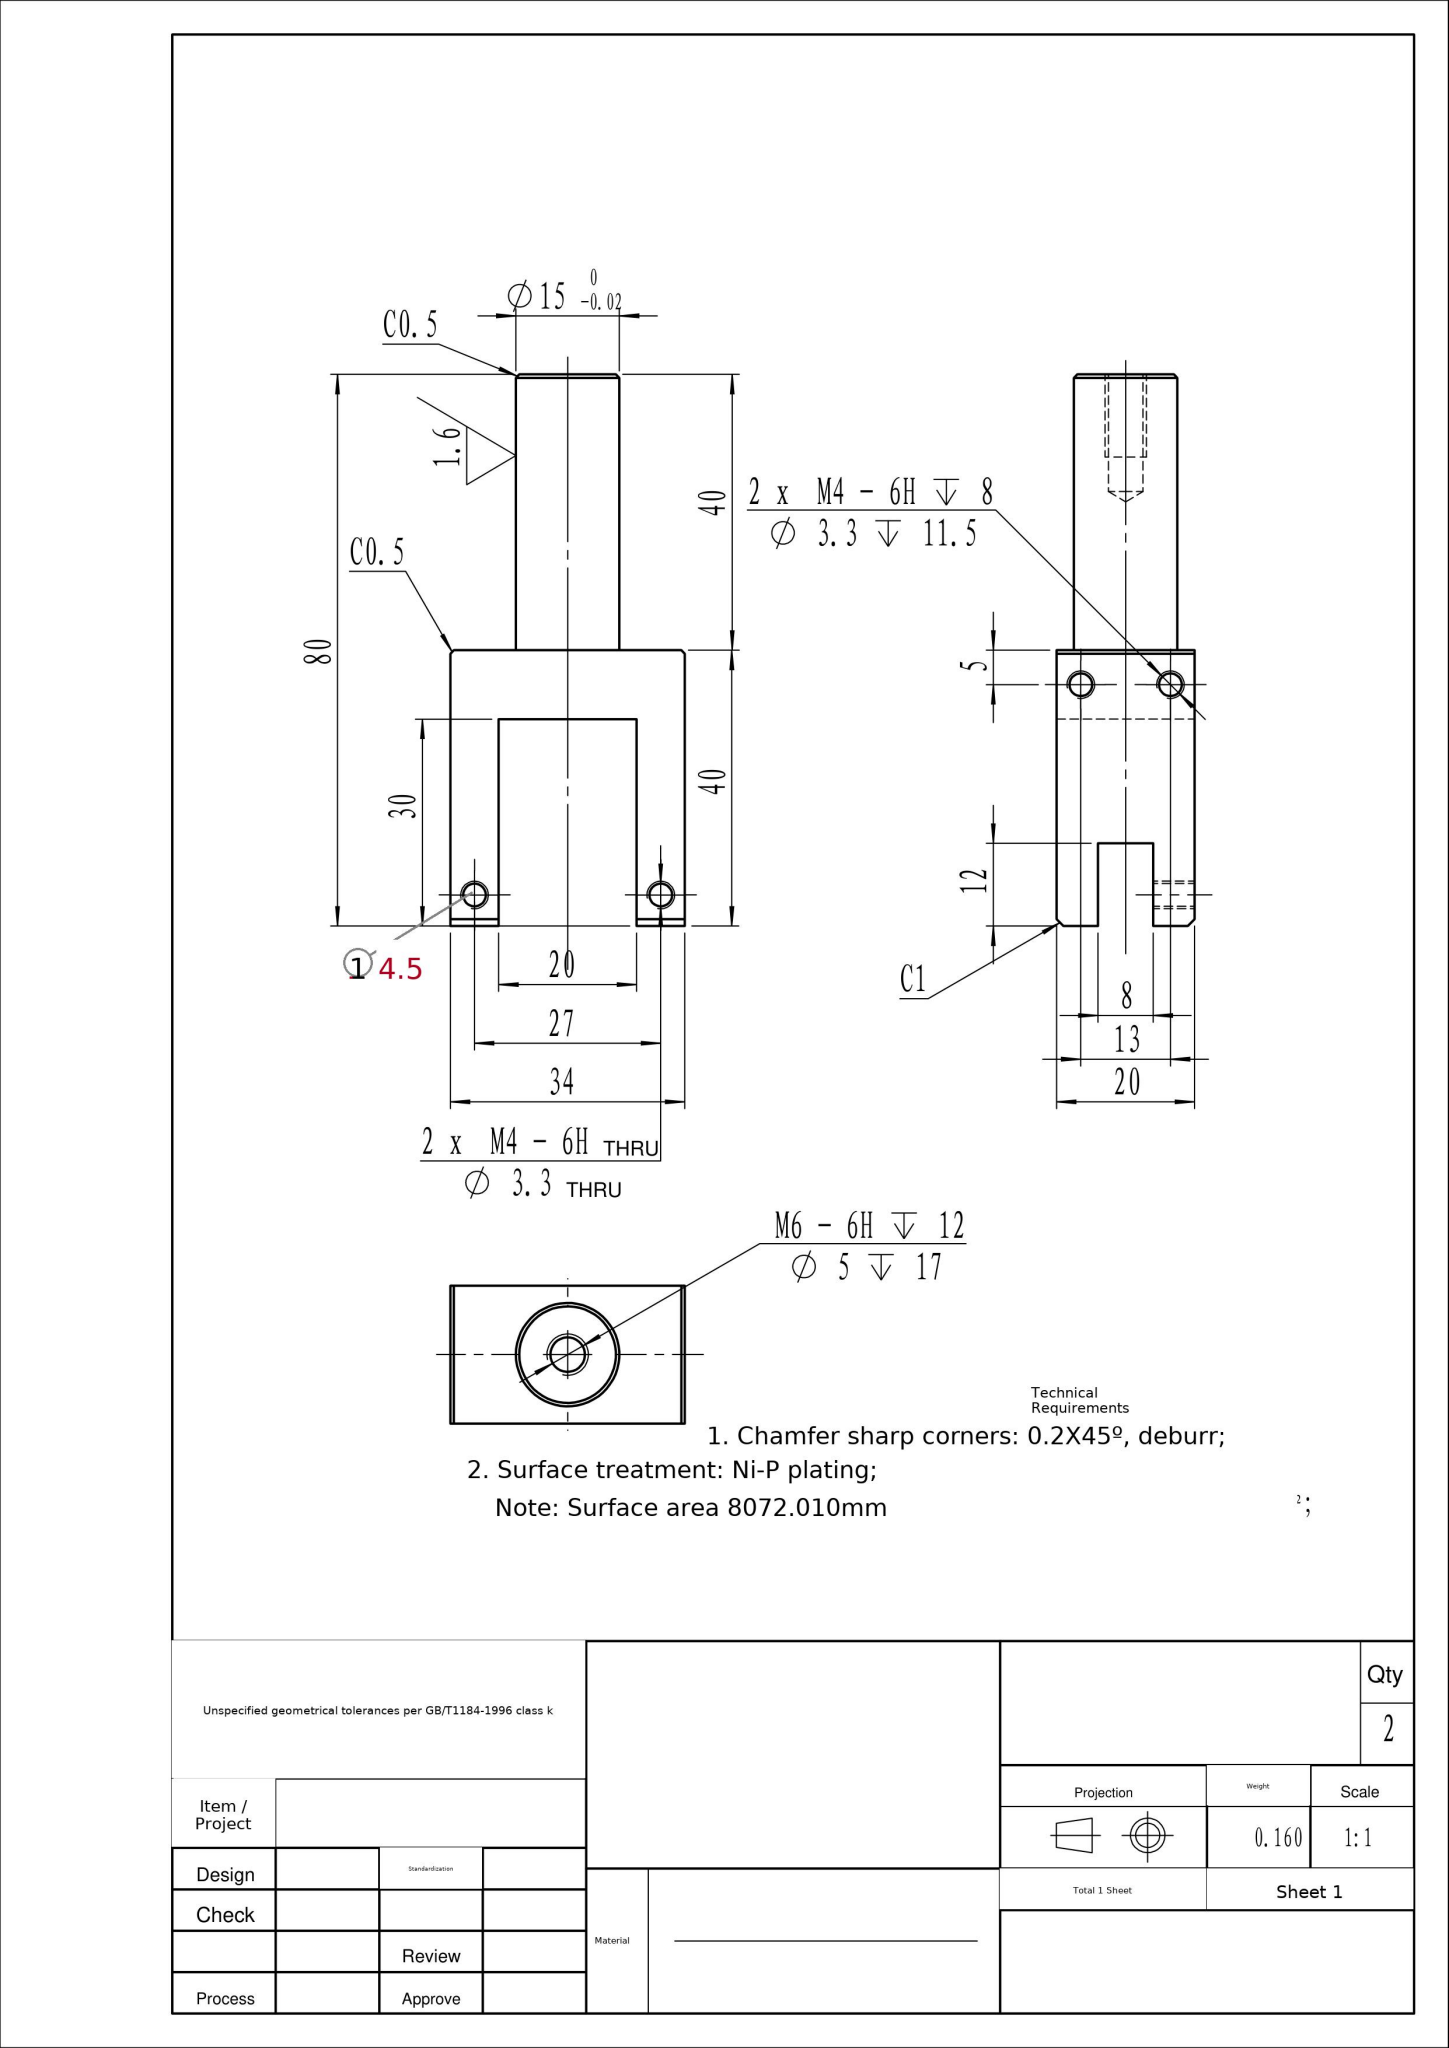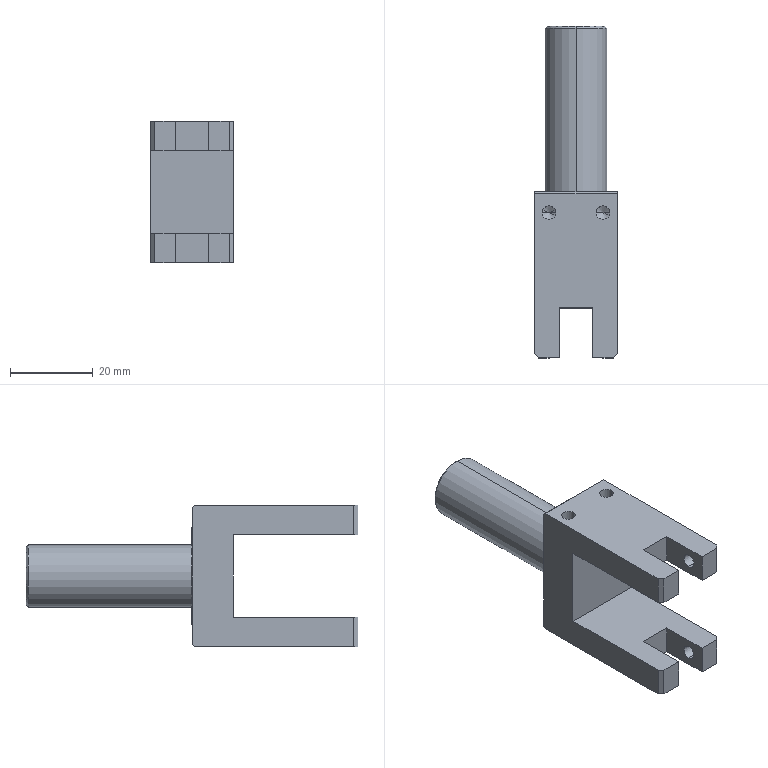Part | SolidWorks | mm | 1 solid | 45 faces | box 20 x 80 x 34 mm | volume 20251 mm3 | plane 25 | cylinder 12 | cone 8 | commonest cylinder face diameters 3.3 x8 5 x2 15 x2
build123d program:
from build123d import *

# Parameters (mm, degrees)
SKETCH1_W             = 34
SKETCH1_H             = 40
BOSS_EXTRUDE1_DEPTH   = 20
SKETCH2_W             = 20
SKETCH2_H             = 30
CUT_EXTRUDE1_DEPTH    = 34
SKETCH3_R             = 7.5
BOSS_EXTRUDE2_DEPTH   = 40
SKETCH5_W             = 8
SKETCH5_H             = 12
CUT_EXTRUDE2_DEPTH    = 72.805
CHAMFER1_SIZE         = 0.5
M4_TAPPED_HOLE1_D     = 3.3
M4_TAPPED_HOLE1_DEPTH = 6
CHAMFER2_SIZE         = 1
CHAMFER3_SIZE         = 0.5
M6_TAPPED_HOLE1_D     = 5
M6_TAPPED_HOLE1_DEPTH = 17
M6_TAPPED_HOLE1_TIP   = 1.502
M4_TAPPED_HOLE2_D     = 3.3
M4_TAPPED_HOLE2_DEPTH = 11.5
M4_TAPPED_HOLE2_TIP   = 0.9914


with BuildPart() as part:
    # Sketch1 → Boss-Extrude1 (new body)
    with BuildSketch(Plane(origin=(0, 0, 0), x_dir=(0, 0, -1), z_dir=(1, 0, 0))):
        Rectangle(SKETCH1_W, SKETCH1_H)
    extrude(amount=BOSS_EXTRUDE1_DEPTH)

    # Sketch2 → Cut-Extrude1 (cut, through all)
    with BuildSketch(Plane(origin=(20, 0, 0), x_dir=(0, 0, -1), z_dir=(1, 0, 0))):
        with Locations((0, -5)):
            Rectangle(SKETCH2_W, SKETCH2_H)
    extrude(amount=-CUT_EXTRUDE1_DEPTH, mode=Mode.SUBTRACT)

    # Sketch3 → Boss-Extrude2 (add)
    with BuildSketch(Plane(origin=(0, 20, 0), x_dir=(1, 0, 0), z_dir=(0, 1, 0))):
        with Locations(Location((10, 0, 0), (0, 0, 90))):
            Circle(SKETCH3_R)
    extrude(amount=BOSS_EXTRUDE2_DEPTH)

    # Sketch5 → Cut-Extrude2 (cut, through all)
    with BuildSketch(Plane.XY.offset(17)):
        with Locations((10, -14)):
            Rectangle(SKETCH5_W, SKETCH5_H)
    extrude(amount=-CUT_EXTRUDE2_DEPTH, mode=Mode.SUBTRACT)

    # Chamfer1
    chamfer1_edges = [part.edges().sort_by_distance(p)[0] for p in [
        (10, 20, 17),
        (10, 20, -17),
    ]]
    chamfer(chamfer1_edges, length=CHAMFER1_SIZE)

    # M4 Tapped Hole1
    with Locations(Plane(origin=(20, 0, 0), x_dir=(0, 0, -1), z_dir=(1, 0, 0))):
        with Locations((-13.5, -15.5), (13.5, -15.5)):
            Hole(M4_TAPPED_HOLE1_D / 2, depth=M4_TAPPED_HOLE1_DEPTH)

    # Chamfer2
    chamfer2_edges = [part.edges().sort_by_distance(p)[0] for p in [
        (20, -20, 13.5),
        (0, -20, -13.5),
        (20, -20, -13.5),
        (0, -20, 13.5),
    ]]
    chamfer(chamfer2_edges, length=CHAMFER2_SIZE)

    # Chamfer3
    chamfer3_edges = [part.edges().sort_by_distance(p)[0] for p in [
        (10, 60, 7.5),
    ]]
    chamfer(chamfer3_edges, length=CHAMFER3_SIZE)

    # M6 Tapped Hole1
    with Locations(Plane(origin=(0, 60, 0), x_dir=(1, 0, 0), z_dir=(0, 1, 0))):
        with Locations((10, 0)):
            Hole(M6_TAPPED_HOLE1_D / 2, depth=M6_TAPPED_HOLE1_DEPTH)
            with Locations((0, 0, -(M6_TAPPED_HOLE1_DEPTH + M6_TAPPED_HOLE1_TIP / 2))):  # 118° drill point
                Cone(0, M6_TAPPED_HOLE1_D / 2, M6_TAPPED_HOLE1_TIP, mode=Mode.SUBTRACT)

    # M4 Tapped Hole2
    with Locations(Plane.XY.offset(17)):
        with Locations((3.5, 15), (16.5, 15)):
            Hole(M4_TAPPED_HOLE2_D / 2, depth=M4_TAPPED_HOLE2_DEPTH)
            with Locations((0, 0, -(M4_TAPPED_HOLE2_DEPTH + M4_TAPPED_HOLE2_TIP / 2))):  # 118° drill point
                Cone(0, M4_TAPPED_HOLE2_D / 2, M4_TAPPED_HOLE2_TIP, mode=Mode.SUBTRACT)


solid = part.part